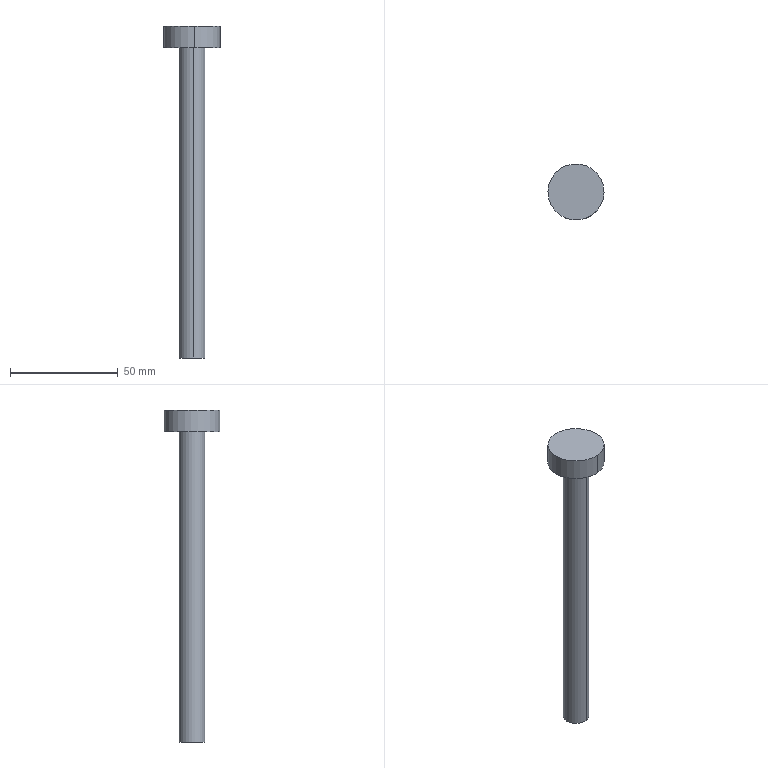Component | SolidWorks | StripAxis-1 | 1 solid | 7 faces | box 26 x 26 x 153.72 mm | volume 21564 mm3 | cylinder 4 | plane 3 | commonest cylinder face diameters 12 x2 26 x2
build123d program:
from build123d import *

# Parameters (mm, degrees)
SKETCH1_R           = 13
BOSS_EXTRUDE1_DEPTH = 10
SKETCH2_R           = 6
BOSS_EXTRUDE2_DEPTH = 143.72


with BuildPart() as part:
    # Sketch1 → Boss-Extrude1 (new body)
    with BuildSketch(Plane.XY):
        with Locations((0, -99.78)):
            Circle(SKETCH1_R)
    extrude(amount=-BOSS_EXTRUDE1_DEPTH)

    # Sketch2 → Boss-Extrude2 (add)
    with BuildSketch(Plane(origin=(0, 0, -10), x_dir=(-1, 0, 0), z_dir=(0, 0, -1))):
        with Locations((0, -99.78)):
            Circle(SKETCH2_R)
    extrude(amount=BOSS_EXTRUDE2_DEPTH)


solid = part.part

# Placed as in the assembly
solid = solid.moved(Location((-266.709, 168.825, 208.72), (0, 0, 0)))
STEP:
#1=COLOUR_RGB('',0.7922,0.8196,0.9333);
#2=FILL_AREA_STYLE_COLOUR('',#1);
#3=FILL_AREA_STYLE('',(#2));
#4=SURFACE_STYLE_FILL_AREA(#3);
#5=SURFACE_SIDE_STYLE('',(#4));
#6=SURFACE_STYLE_USAGE(.BOTH.,#5);
#7=PRESENTATION_STYLE_ASSIGNMENT((#6));
#8=CARTESIAN_POINT('',(-10.523,2.953,2.165));
#9=VERTEX_POINT('',#8);
#10=CARTESIAN_POINT('',(-10.478,2.483,2.165));
#11=VERTEX_POINT('',#10);
#12=CARTESIAN_POINT('',(-10.5,2.718,2.165));
#13=DIRECTION('',(0.,0.,-1.));
#14=DIRECTION('',(-0.09661,0.9953,0.));
#15=AXIS2_PLACEMENT_3D('',#12,#13,#14);
#16=CIRCLE('',#15,0.2362);
#17=EDGE_CURVE('',#9,#11,#16,.T.);
#18=ORIENTED_EDGE('',*,*,#17,.F.);
#19=CARTESIAN_POINT('',(-10.523,2.953,7.824));
#20=VERTEX_POINT('',#19);
#21=CARTESIAN_POINT('',(-10.523,2.953,2.165));
#22=DIRECTION('',(-0.,-0.,1.));
#23=VECTOR('',#22,39.37);
#24=LINE('',#21,#23);
#25=EDGE_CURVE('',#9,#20,#24,.T.);
#26=ORIENTED_EDGE('',*,*,#25,.T.);
#27=CARTESIAN_POINT('',(-10.478,2.483,7.824));
#28=VERTEX_POINT('',#27);
#29=CARTESIAN_POINT('',(-10.5,2.718,7.824));
#30=DIRECTION('',(0.,0.,-1.));
#31=DIRECTION('',(-0.09661,0.9953,0.));
#32=AXIS2_PLACEMENT_3D('',#29,#30,#31);
#33=CIRCLE('',#32,0.2362);
#34=EDGE_CURVE('',#20,#28,#33,.T.);
#35=ORIENTED_EDGE('',*,*,#34,.T.);
#36=CARTESIAN_POINT('',(-10.478,2.483,2.165));
#37=DIRECTION('',(-0.,-0.,1.));
#38=VECTOR('',#37,39.37);
#39=LINE('',#36,#38);
#40=EDGE_CURVE('',#11,#28,#39,.T.);
#41=ORIENTED_EDGE('',*,*,#40,.F.);
#42=EDGE_LOOP('',(#18,#26,#35,#41));
#43=FACE_OUTER_BOUND('',#42,.T.);
#44=CARTESIAN_POINT('',(-10.5,2.718,2.165));
#45=DIRECTION('',(-0.,-0.,1.));
#46=DIRECTION('',(0.09661,-0.9953,0.));
#47=AXIS2_PLACEMENT_3D('',#44,#45,#46);
#48=CYLINDRICAL_SURFACE('',#47,0.2362);
#49=ADVANCED_FACE('',(#43),#48,.T.);
#50=CARTESIAN_POINT('',(-10.451,2.209,7.824));
#51=VERTEX_POINT('',#50);
#52=CARTESIAN_POINT('',(-10.55,3.228,7.824));
#53=VERTEX_POINT('',#52);
#54=CARTESIAN_POINT('',(-10.5,2.718,7.824));
#55=DIRECTION('',(-0.,-0.,1.));
#56=DIRECTION('',(0.09661,-0.9953,0.));
#57=AXIS2_PLACEMENT_3D('',#54,#55,#56);
#58=CIRCLE('',#57,0.5118);
#59=EDGE_CURVE('',#51,#53,#58,.T.);
#60=ORIENTED_EDGE('',*,*,#59,.T.);
#61=CARTESIAN_POINT('',(-10.55,3.228,8.217));
#62=VERTEX_POINT('',#61);
#63=CARTESIAN_POINT('',(-10.55,3.228,7.824));
#64=DIRECTION('',(-0.,-0.,1.));
#65=VECTOR('',#64,39.37);
#66=LINE('',#63,#65);
#67=EDGE_CURVE('',#53,#62,#66,.T.);
#68=ORIENTED_EDGE('',*,*,#67,.T.);
#69=CARTESIAN_POINT('',(-10.451,2.209,8.217));
#70=VERTEX_POINT('',#69);
#71=CARTESIAN_POINT('',(-10.5,2.718,8.217));
#72=DIRECTION('',(-0.,-0.,1.));
#73=DIRECTION('',(0.09661,-0.9953,0.));
#74=AXIS2_PLACEMENT_3D('',#71,#72,#73);
#75=CIRCLE('',#74,0.5118);
#76=EDGE_CURVE('',#70,#62,#75,.T.);
#77=ORIENTED_EDGE('',*,*,#76,.F.);
#78=CARTESIAN_POINT('',(-10.451,2.209,7.824));
#79=DIRECTION('',(-0.,-0.,1.));
#80=VECTOR('',#79,39.37);
#81=LINE('',#78,#80);
#82=EDGE_CURVE('',#51,#70,#81,.T.);
#83=ORIENTED_EDGE('',*,*,#82,.F.);
#84=EDGE_LOOP('',(#60,#68,#77,#83));
#85=FACE_OUTER_BOUND('',#84,.T.);
#86=CARTESIAN_POINT('',(-10.5,2.718,7.824));
#87=DIRECTION('',(-0.,-0.,1.));
#88=DIRECTION('',(0.09661,-0.9953,0.));
#89=AXIS2_PLACEMENT_3D('',#86,#87,#88);
#90=CYLINDRICAL_SURFACE('',#89,0.5118);
#91=ADVANCED_FACE('',(#85),#90,.T.);
#92=ORIENTED_EDGE('',*,*,#67,.F.);
#93=CARTESIAN_POINT('',(-10.5,2.718,7.824));
#94=DIRECTION('',(-0.,-0.,1.));
#95=DIRECTION('',(0.09661,-0.9953,0.));
#96=AXIS2_PLACEMENT_3D('',#93,#94,#95);
#97=CIRCLE('',#96,0.5118);
#98=EDGE_CURVE('',#53,#51,#97,.T.);
#99=ORIENTED_EDGE('',*,*,#98,.T.);
#100=ORIENTED_EDGE('',*,*,#82,.T.);
#101=CARTESIAN_POINT('',(-10.5,2.718,8.217));
#102=DIRECTION('',(-0.,-0.,1.));
#103=DIRECTION('',(0.09661,-0.9953,0.));
#104=AXIS2_PLACEMENT_3D('',#101,#102,#103);
#105=CIRCLE('',#104,0.5118);
#106=EDGE_CURVE('',#62,#70,#105,.T.);
#107=ORIENTED_EDGE('',*,*,#106,.F.);
#108=EDGE_LOOP('',(#92,#99,#100,#107));
#109=FACE_OUTER_BOUND('',#108,.T.);
#110=CARTESIAN_POINT('',(-10.5,2.718,7.824));
#111=DIRECTION('',(-0.,-0.,1.));
#112=DIRECTION('',(0.09661,-0.9953,0.));
#113=AXIS2_PLACEMENT_3D('',#110,#111,#112);
#114=CYLINDRICAL_SURFACE('',#113,0.5118);
#115=ADVANCED_FACE('',(#109),#114,.T.);
#116=CARTESIAN_POINT('',(-10.5,2.718,7.824));
#117=DIRECTION('',(0.,0.,-1.));
#118=DIRECTION('',(-0.09661,0.9953,0.));
#119=AXIS2_PLACEMENT_3D('',#116,#117,#118);
#120=CIRCLE('',#119,0.2362);
#121=EDGE_CURVE('',#28,#20,#120,.T.);
#122=ORIENTED_EDGE('',*,*,#121,.F.);
#123=ORIENTED_EDGE('',*,*,#34,.F.);
#124=EDGE_LOOP('',(#122,#123));
#125=FACE_BOUND('',#124,.T.);
#126=ORIENTED_EDGE('',*,*,#59,.F.);
#127=ORIENTED_EDGE('',*,*,#98,.F.);
#128=EDGE_LOOP('',(#126,#127));
#129=FACE_OUTER_BOUND('',#128,.T.);
#130=CARTESIAN_POINT('',(-10.5,2.718,7.824));
#131=DIRECTION('',(-0.,-0.,1.));
#132=DIRECTION('',(0.09661,-0.9953,-0.));
#133=AXIS2_PLACEMENT_3D('',#130,#131,#132);
#134=PLANE('',#133);
#135=ADVANCED_FACE('',(#125,#129),#134,.F.);
#136=ORIENTED_EDGE('',*,*,#76,.T.);
#137=ORIENTED_EDGE('',*,*,#106,.T.);
#138=EDGE_LOOP('',(#136,#137));
#139=FACE_OUTER_BOUND('',#138,.T.);
#140=CARTESIAN_POINT('',(-10.5,2.718,8.217));
#141=DIRECTION('',(-0.,-0.,1.));
#142=DIRECTION('',(0.09661,-0.9953,-0.));
#143=AXIS2_PLACEMENT_3D('',#140,#141,#142);
#144=PLANE('',#143);
#145=ADVANCED_FACE('',(#139),#144,.T.);
#146=ORIENTED_EDGE('',*,*,#25,.F.);
#147=CARTESIAN_POINT('',(-10.5,2.718,2.165));
#148=DIRECTION('',(0.,0.,-1.));
#149=DIRECTION('',(-0.09661,0.9953,0.));
#150=AXIS2_PLACEMENT_3D('',#147,#148,#149);
#151=CIRCLE('',#150,0.2362);
#152=EDGE_CURVE('',#11,#9,#151,.T.);
#153=ORIENTED_EDGE('',*,*,#152,.F.);
#154=ORIENTED_EDGE('',*,*,#40,.T.);
#155=ORIENTED_EDGE('',*,*,#121,.T.);
#156=EDGE_LOOP('',(#146,#153,#154,#155));
#157=FACE_OUTER_BOUND('',#156,.T.);
#158=CARTESIAN_POINT('',(-10.5,2.718,2.165));
#159=DIRECTION('',(-0.,-0.,1.));
#160=DIRECTION('',(0.09661,-0.9953,0.));
#161=AXIS2_PLACEMENT_3D('',#158,#159,#160);
#162=CYLINDRICAL_SURFACE('',#161,0.2362);
#163=ADVANCED_FACE('',(#157),#162,.T.);
#164=ORIENTED_EDGE('',*,*,#152,.T.);
#165=ORIENTED_EDGE('',*,*,#17,.T.);
#166=EDGE_LOOP('',(#164,#165));
#167=FACE_OUTER_BOUND('',#166,.T.);
#168=CARTESIAN_POINT('',(-10.5,2.718,2.165));
#169=DIRECTION('',(0.,0.,-1.));
#170=DIRECTION('',(-0.09661,0.9953,0.));
#171=AXIS2_PLACEMENT_3D('',#168,#169,#170);
#172=PLANE('',#171);
#173=ADVANCED_FACE('',(#167),#172,.T.);
#174=CLOSED_SHELL('',(#49,#91,#115,#135,#145,#163,#173));
#175=MANIFOLD_SOLID_BREP('',#174);
#176=STYLED_ITEM('',(#7),#175);
#177=PRESENTATION_LAYER_ASSIGNMENT('','',(#176));
#178=(LENGTH_UNIT()NAMED_UNIT(*)SI_UNIT($,.METRE.));
#179=LENGTH_MEASURE_WITH_UNIT(LENGTH_MEASURE(0.0254),#178);
#180=DIMENSIONAL_EXPONENTS(1.,0.,0.,0.,0.,0.,0.);
#181=(CONVERSION_BASED_UNIT('',#179)LENGTH_UNIT()NAMED_UNIT(#180));
#182=UNCERTAINTY_MEASURE_WITH_UNIT(LENGTH_MEASURE(0.00001),#181,'','');
#183=(NAMED_UNIT(*)PLANE_ANGLE_UNIT()SI_UNIT($,.RADIAN.));
#184=(NAMED_UNIT(*)SI_UNIT($,.STERADIAN.)SOLID_ANGLE_UNIT());
#185=(GEOMETRIC_REPRESENTATION_CONTEXT(3)GLOBAL_UNCERTAINTY_ASSIGNED_CONTEXT((#182))GLOBAL_UNIT_ASSIGNED_CONTEXT((#181,#183,#184))REPRESENTATION_CONTEXT('',''));
#186=MECHANICAL_DESIGN_GEOMETRIC_PRESENTATION_REPRESENTATION('',(#176),#185);
#187=CARTESIAN_POINT('',(0.,0.,0.));
#188=DIRECTION('',(0.,0.,1.));
#189=DIRECTION('',(1.,0.,0.));
#190=AXIS2_PLACEMENT_3D('',#187,#188,#189);
#191=(LENGTH_UNIT()NAMED_UNIT(*)SI_UNIT($,.METRE.));
#192=LENGTH_MEASURE_WITH_UNIT(LENGTH_MEASURE(0.0254),#191);
#193=DIMENSIONAL_EXPONENTS(1.,0.,0.,0.,0.,0.,0.);
#194=(CONVERSION_BASED_UNIT('',#192)LENGTH_UNIT()NAMED_UNIT(#193));
#195=UNCERTAINTY_MEASURE_WITH_UNIT(LENGTH_MEASURE(0.00001),#194,'','');
#196=(NAMED_UNIT(*)PLANE_ANGLE_UNIT()SI_UNIT($,.RADIAN.));
#197=(NAMED_UNIT(*)SI_UNIT($,.STERADIAN.)SOLID_ANGLE_UNIT());
#198=(GEOMETRIC_REPRESENTATION_CONTEXT(3)GLOBAL_UNCERTAINTY_ASSIGNED_CONTEXT((#195))GLOBAL_UNIT_ASSIGNED_CONTEXT((#194,#196,#197))REPRESENTATION_CONTEXT('',''));
#199=ADVANCED_BREP_SHAPE_REPRESENTATION('',(#175,#190),#198);